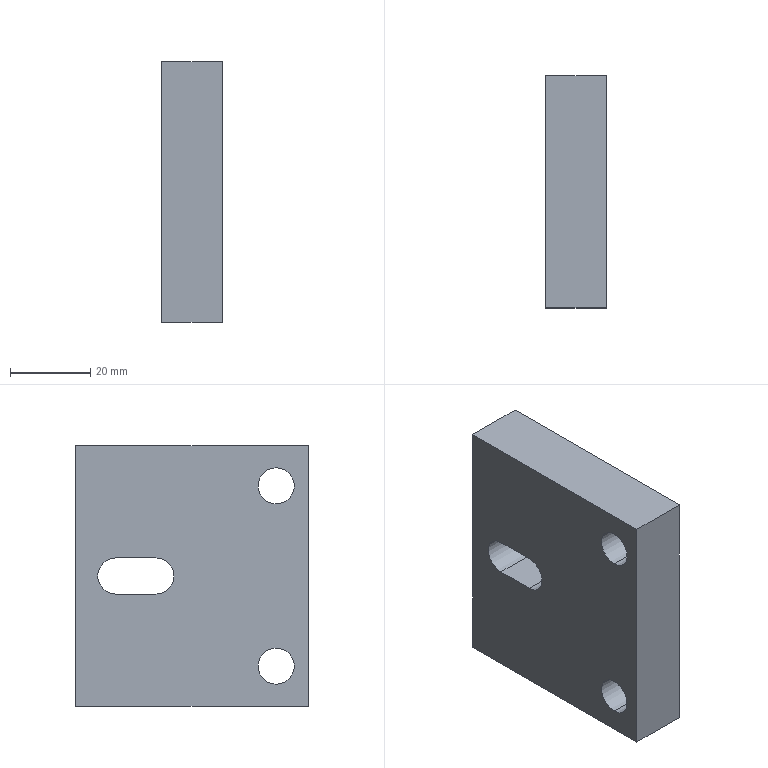Component | SolidWorks | TractionTensionPlate-2 | 1 solid | 14 faces | box 15 x 58 x 65 mm | volume 52337 mm3 | plane 8 | cylinder 6 | commonest cylinder face diameters 9 x6
build123d program:
from build123d import *

# Parameters (mm, degrees)
SKETCH1_W      = 65
SKETCH1_H      = 58
SKETCH1_R      = 4.5
EXTRUDE1_DEPTH = 15


with BuildPart() as part:
    # Sketch1 → Extrude1 (new body)
    with BuildSketch(Plane.XY):
        Rectangle(SKETCH1_W, SKETCH1_H)
        with Locations((-22.5, -21)):
            Circle(SKETCH1_R, mode=Mode.SUBTRACT)
        with Locations((22.5, -21)):
            Circle(SKETCH1_R, mode=Mode.SUBTRACT)
        with BuildLine():
            Line((-4.5, 19), (-4.5, 9))
            ThreePointArc((-4.5, 9), (0, 4.5), (4.5, 9))
            Line((4.5, 9), (4.5, 19))
            ThreePointArc((4.5, 19), (0, 23.5), (-4.5, 19))
        make_face(mode=Mode.SUBTRACT)
    extrude(amount=EXTRUDE1_DEPTH)


solid = part.part

# Placed as in the assembly
solid = solid.moved(Location((50.216, 516.983, 59.606), (0, 90, 0)))
STEP:
#1=CARTESIAN_POINT('',(2.568,19.527,1.638));
#2=VERTEX_POINT('',#1);
#3=CARTESIAN_POINT('',(2.568,19.527,1.284));
#4=VERTEX_POINT('',#3);
#5=CARTESIAN_POINT('',(2.568,19.527,1.461));
#6=DIRECTION('',(1.,0.,0.));
#7=DIRECTION('',(0.,0.,-1.));
#8=AXIS2_PLACEMENT_3D('',#5,#6,#7);
#9=CIRCLE('',#8,0.1772);
#10=EDGE_CURVE('',#2,#4,#9,.T.);
#11=ORIENTED_EDGE('',*,*,#10,.T.);
#12=CARTESIAN_POINT('',(1.977,19.527,1.284));
#13=VERTEX_POINT('',#12);
#14=CARTESIAN_POINT('',(2.568,19.527,1.284));
#15=DIRECTION('',(-1.,0.,0.));
#16=VECTOR('',#15,39.37);
#17=LINE('',#14,#16);
#18=EDGE_CURVE('',#4,#13,#17,.T.);
#19=ORIENTED_EDGE('',*,*,#18,.T.);
#20=CARTESIAN_POINT('',(1.977,19.527,1.638));
#21=VERTEX_POINT('',#20);
#22=CARTESIAN_POINT('',(1.977,19.527,1.461));
#23=DIRECTION('',(1.,0.,0.));
#24=DIRECTION('',(0.,0.,-1.));
#25=AXIS2_PLACEMENT_3D('',#22,#23,#24);
#26=CIRCLE('',#25,0.1772);
#27=EDGE_CURVE('',#21,#13,#26,.T.);
#28=ORIENTED_EDGE('',*,*,#27,.F.);
#29=CARTESIAN_POINT('',(2.568,19.527,1.638));
#30=DIRECTION('',(-1.,0.,0.));
#31=VECTOR('',#30,39.37);
#32=LINE('',#29,#31);
#33=EDGE_CURVE('',#2,#21,#32,.T.);
#34=ORIENTED_EDGE('',*,*,#33,.F.);
#35=EDGE_LOOP('',(#11,#19,#28,#34));
#36=FACE_OUTER_BOUND('',#35,.T.);
#37=CARTESIAN_POINT('',(2.568,19.527,1.461));
#38=DIRECTION('',(-1.,0.,0.));
#39=DIRECTION('',(0.,0.,1.));
#40=AXIS2_PLACEMENT_3D('',#37,#38,#39);
#41=CYLINDRICAL_SURFACE('',#40,0.1772);
#42=ADVANCED_FACE('',(#36),#41,.F.);
#43=CARTESIAN_POINT('',(2.568,19.527,3.41));
#44=VERTEX_POINT('',#43);
#45=CARTESIAN_POINT('',(2.568,19.527,3.055));
#46=VERTEX_POINT('',#45);
#47=CARTESIAN_POINT('',(2.568,19.527,3.233));
#48=DIRECTION('',(1.,0.,0.));
#49=DIRECTION('',(0.,0.,-1.));
#50=AXIS2_PLACEMENT_3D('',#47,#48,#49);
#51=CIRCLE('',#50,0.1772);
#52=EDGE_CURVE('',#44,#46,#51,.T.);
#53=ORIENTED_EDGE('',*,*,#52,.T.);
#54=CARTESIAN_POINT('',(1.977,19.527,3.055));
#55=VERTEX_POINT('',#54);
#56=CARTESIAN_POINT('',(2.568,19.527,3.055));
#57=DIRECTION('',(-1.,0.,0.));
#58=VECTOR('',#57,39.37);
#59=LINE('',#56,#58);
#60=EDGE_CURVE('',#46,#55,#59,.T.);
#61=ORIENTED_EDGE('',*,*,#60,.T.);
#62=CARTESIAN_POINT('',(1.977,19.527,3.41));
#63=VERTEX_POINT('',#62);
#64=CARTESIAN_POINT('',(1.977,19.527,3.233));
#65=DIRECTION('',(1.,0.,0.));
#66=DIRECTION('',(0.,0.,-1.));
#67=AXIS2_PLACEMENT_3D('',#64,#65,#66);
#68=CIRCLE('',#67,0.1772);
#69=EDGE_CURVE('',#63,#55,#68,.T.);
#70=ORIENTED_EDGE('',*,*,#69,.F.);
#71=CARTESIAN_POINT('',(2.568,19.527,3.41));
#72=DIRECTION('',(-1.,0.,0.));
#73=VECTOR('',#72,39.37);
#74=LINE('',#71,#73);
#75=EDGE_CURVE('',#44,#63,#74,.T.);
#76=ORIENTED_EDGE('',*,*,#75,.F.);
#77=EDGE_LOOP('',(#53,#61,#70,#76));
#78=FACE_OUTER_BOUND('',#77,.T.);
#79=CARTESIAN_POINT('',(2.568,19.527,3.233));
#80=DIRECTION('',(-1.,0.,0.));
#81=DIRECTION('',(0.,0.,1.));
#82=AXIS2_PLACEMENT_3D('',#79,#80,#81);
#83=CYLINDRICAL_SURFACE('',#82,0.1772);
#84=ADVANCED_FACE('',(#78),#83,.F.);
#85=ORIENTED_EDGE('',*,*,#52,.F.);
#86=CARTESIAN_POINT('',(2.568,19.527,3.233));
#87=DIRECTION('',(1.,0.,0.));
#88=DIRECTION('',(0.,0.,-1.));
#89=AXIS2_PLACEMENT_3D('',#86,#87,#88);
#90=CIRCLE('',#89,0.1772);
#91=EDGE_CURVE('',#46,#44,#90,.T.);
#92=ORIENTED_EDGE('',*,*,#91,.F.);
#93=EDGE_LOOP('',(#85,#92));
#94=FACE_BOUND('',#93,.T.);
#95=CARTESIAN_POINT('',(2.568,21.495,3.626));
#96=VERTEX_POINT('',#95);
#97=CARTESIAN_POINT('',(2.568,19.212,3.626));
#98=VERTEX_POINT('',#97);
#99=CARTESIAN_POINT('',(2.568,21.495,3.626));
#100=DIRECTION('',(0.,-1.,0.));
#101=VECTOR('',#100,39.37);
#102=LINE('',#99,#101);
#103=EDGE_CURVE('',#96,#98,#102,.T.);
#104=ORIENTED_EDGE('',*,*,#103,.T.);
#105=CARTESIAN_POINT('',(2.568,19.212,1.067));
#106=VERTEX_POINT('',#105);
#107=CARTESIAN_POINT('',(2.568,19.212,3.626));
#108=DIRECTION('',(0.,0.,-1.));
#109=VECTOR('',#108,39.37);
#110=LINE('',#107,#109);
#111=EDGE_CURVE('',#98,#106,#110,.T.);
#112=ORIENTED_EDGE('',*,*,#111,.T.);
#113=CARTESIAN_POINT('',(2.568,21.495,1.067));
#114=VERTEX_POINT('',#113);
#115=CARTESIAN_POINT('',(2.568,21.495,1.067));
#116=DIRECTION('',(0.,1.,0.));
#117=VECTOR('',#116,39.37);
#118=LINE('',#115,#117);
#119=EDGE_CURVE('',#106,#114,#118,.T.);
#120=ORIENTED_EDGE('',*,*,#119,.T.);
#121=CARTESIAN_POINT('',(2.568,21.495,3.626));
#122=DIRECTION('',(0.,0.,1.));
#123=VECTOR('',#122,39.37);
#124=LINE('',#121,#123);
#125=EDGE_CURVE('',#114,#96,#124,.T.);
#126=ORIENTED_EDGE('',*,*,#125,.T.);
#127=EDGE_LOOP('',(#104,#112,#120,#126));
#128=FACE_OUTER_BOUND('',#127,.T.);
#129=ORIENTED_EDGE('',*,*,#10,.F.);
#130=CARTESIAN_POINT('',(2.568,19.527,1.461));
#131=DIRECTION('',(1.,0.,0.));
#132=DIRECTION('',(0.,0.,-1.));
#133=AXIS2_PLACEMENT_3D('',#130,#131,#132);
#134=CIRCLE('',#133,0.1772);
#135=EDGE_CURVE('',#4,#2,#134,.T.);
#136=ORIENTED_EDGE('',*,*,#135,.F.);
#137=EDGE_LOOP('',(#129,#136));
#138=FACE_BOUND('',#137,.T.);
#139=CARTESIAN_POINT('',(2.568,21.102,2.524));
#140=VERTEX_POINT('',#139);
#141=CARTESIAN_POINT('',(2.568,20.708,2.524));
#142=VERTEX_POINT('',#141);
#143=CARTESIAN_POINT('',(2.568,21.102,2.524));
#144=DIRECTION('',(0.,-1.,0.));
#145=VECTOR('',#144,39.37);
#146=LINE('',#143,#145);
#147=EDGE_CURVE('',#140,#142,#146,.T.);
#148=ORIENTED_EDGE('',*,*,#147,.F.);
#149=CARTESIAN_POINT('',(2.568,21.102,2.17));
#150=VERTEX_POINT('',#149);
#151=CARTESIAN_POINT('',(2.568,21.102,2.347));
#152=DIRECTION('',(1.,0.,0.));
#153=DIRECTION('',(0.,0.,-1.));
#154=AXIS2_PLACEMENT_3D('',#151,#152,#153);
#155=CIRCLE('',#154,0.1772);
#156=EDGE_CURVE('',#150,#140,#155,.T.);
#157=ORIENTED_EDGE('',*,*,#156,.F.);
#158=CARTESIAN_POINT('',(2.568,20.708,2.17));
#159=VERTEX_POINT('',#158);
#160=CARTESIAN_POINT('',(2.568,21.102,2.17));
#161=DIRECTION('',(0.,1.,0.));
#162=VECTOR('',#161,39.37);
#163=LINE('',#160,#162);
#164=EDGE_CURVE('',#159,#150,#163,.T.);
#165=ORIENTED_EDGE('',*,*,#164,.F.);
#166=CARTESIAN_POINT('',(2.568,20.708,2.347));
#167=DIRECTION('',(1.,0.,0.));
#168=DIRECTION('',(0.,0.,-1.));
#169=AXIS2_PLACEMENT_3D('',#166,#167,#168);
#170=CIRCLE('',#169,0.1772);
#171=EDGE_CURVE('',#142,#159,#170,.T.);
#172=ORIENTED_EDGE('',*,*,#171,.F.);
#173=EDGE_LOOP('',(#148,#157,#165,#172));
#174=FACE_BOUND('',#173,.T.);
#175=CARTESIAN_POINT('',(2.568,19.212,3.626));
#176=DIRECTION('',(1.,0.,0.));
#177=DIRECTION('',(0.,0.,-1.));
#178=AXIS2_PLACEMENT_3D('',#175,#176,#177);
#179=PLANE('',#178);
#180=ADVANCED_FACE('',(#94,#128,#138,#174),#179,.T.);
#181=ORIENTED_EDGE('',*,*,#27,.T.);
#182=CARTESIAN_POINT('',(1.977,19.527,1.461));
#183=DIRECTION('',(1.,0.,0.));
#184=DIRECTION('',(0.,0.,-1.));
#185=AXIS2_PLACEMENT_3D('',#182,#183,#184);
#186=CIRCLE('',#185,0.1772);
#187=EDGE_CURVE('',#13,#21,#186,.T.);
#188=ORIENTED_EDGE('',*,*,#187,.T.);
#189=EDGE_LOOP('',(#181,#188));
#190=FACE_BOUND('',#189,.T.);
#191=ORIENTED_EDGE('',*,*,#69,.T.);
#192=CARTESIAN_POINT('',(1.977,19.527,3.233));
#193=DIRECTION('',(1.,0.,0.));
#194=DIRECTION('',(0.,0.,-1.));
#195=AXIS2_PLACEMENT_3D('',#192,#193,#194);
#196=CIRCLE('',#195,0.1772);
#197=EDGE_CURVE('',#55,#63,#196,.T.);
#198=ORIENTED_EDGE('',*,*,#197,.T.);
#199=EDGE_LOOP('',(#191,#198));
#200=FACE_BOUND('',#199,.T.);
#201=CARTESIAN_POINT('',(1.977,21.495,3.626));
#202=VERTEX_POINT('',#201);
#203=CARTESIAN_POINT('',(1.977,19.212,3.626));
#204=VERTEX_POINT('',#203);
#205=CARTESIAN_POINT('',(1.977,21.495,3.626));
#206=DIRECTION('',(0.,-1.,0.));
#207=VECTOR('',#206,39.37);
#208=LINE('',#205,#207);
#209=EDGE_CURVE('',#202,#204,#208,.T.);
#210=ORIENTED_EDGE('',*,*,#209,.F.);
#211=CARTESIAN_POINT('',(1.977,21.495,1.067));
#212=VERTEX_POINT('',#211);
#213=CARTESIAN_POINT('',(1.977,21.495,3.626));
#214=DIRECTION('',(0.,0.,1.));
#215=VECTOR('',#214,39.37);
#216=LINE('',#213,#215);
#217=EDGE_CURVE('',#212,#202,#216,.T.);
#218=ORIENTED_EDGE('',*,*,#217,.F.);
#219=CARTESIAN_POINT('',(1.977,19.212,1.067));
#220=VERTEX_POINT('',#219);
#221=CARTESIAN_POINT('',(1.977,21.495,1.067));
#222=DIRECTION('',(0.,1.,0.));
#223=VECTOR('',#222,39.37);
#224=LINE('',#221,#223);
#225=EDGE_CURVE('',#220,#212,#224,.T.);
#226=ORIENTED_EDGE('',*,*,#225,.F.);
#227=CARTESIAN_POINT('',(1.977,19.212,3.626));
#228=DIRECTION('',(0.,0.,-1.));
#229=VECTOR('',#228,39.37);
#230=LINE('',#227,#229);
#231=EDGE_CURVE('',#204,#220,#230,.T.);
#232=ORIENTED_EDGE('',*,*,#231,.F.);
#233=EDGE_LOOP('',(#210,#218,#226,#232));
#234=FACE_OUTER_BOUND('',#233,.T.);
#235=CARTESIAN_POINT('',(1.977,21.102,2.17));
#236=VERTEX_POINT('',#235);
#237=CARTESIAN_POINT('',(1.977,21.102,2.524));
#238=VERTEX_POINT('',#237);
#239=CARTESIAN_POINT('',(1.977,21.102,2.347));
#240=DIRECTION('',(1.,0.,0.));
#241=DIRECTION('',(0.,0.,-1.));
#242=AXIS2_PLACEMENT_3D('',#239,#240,#241);
#243=CIRCLE('',#242,0.1772);
#244=EDGE_CURVE('',#236,#238,#243,.T.);
#245=ORIENTED_EDGE('',*,*,#244,.T.);
#246=CARTESIAN_POINT('',(1.977,20.708,2.524));
#247=VERTEX_POINT('',#246);
#248=CARTESIAN_POINT('',(1.977,21.102,2.524));
#249=DIRECTION('',(0.,-1.,0.));
#250=VECTOR('',#249,39.37);
#251=LINE('',#248,#250);
#252=EDGE_CURVE('',#238,#247,#251,.T.);
#253=ORIENTED_EDGE('',*,*,#252,.T.);
#254=CARTESIAN_POINT('',(1.977,20.708,2.17));
#255=VERTEX_POINT('',#254);
#256=CARTESIAN_POINT('',(1.977,20.708,2.347));
#257=DIRECTION('',(1.,0.,0.));
#258=DIRECTION('',(0.,0.,-1.));
#259=AXIS2_PLACEMENT_3D('',#256,#257,#258);
#260=CIRCLE('',#259,0.1772);
#261=EDGE_CURVE('',#247,#255,#260,.T.);
#262=ORIENTED_EDGE('',*,*,#261,.T.);
#263=CARTESIAN_POINT('',(1.977,21.102,2.17));
#264=DIRECTION('',(0.,1.,0.));
#265=VECTOR('',#264,39.37);
#266=LINE('',#263,#265);
#267=EDGE_CURVE('',#255,#236,#266,.T.);
#268=ORIENTED_EDGE('',*,*,#267,.T.);
#269=EDGE_LOOP('',(#245,#253,#262,#268));
#270=FACE_BOUND('',#269,.T.);
#271=CARTESIAN_POINT('',(1.977,19.212,3.626));
#272=DIRECTION('',(1.,0.,0.));
#273=DIRECTION('',(0.,0.,-1.));
#274=AXIS2_PLACEMENT_3D('',#271,#272,#273);
#275=PLANE('',#274);
#276=ADVANCED_FACE('',(#190,#200,#234,#270),#275,.F.);
#277=ORIENTED_EDGE('',*,*,#209,.T.);
#278=CARTESIAN_POINT('',(2.568,19.212,3.626));
#279=DIRECTION('',(-1.,0.,0.));
#280=VECTOR('',#279,39.37);
#281=LINE('',#278,#280);
#282=EDGE_CURVE('',#98,#204,#281,.T.);
#283=ORIENTED_EDGE('',*,*,#282,.F.);
#284=ORIENTED_EDGE('',*,*,#103,.F.);
#285=CARTESIAN_POINT('',(2.568,21.495,3.626));
#286=DIRECTION('',(-1.,0.,0.));
#287=VECTOR('',#286,39.37);
#288=LINE('',#285,#287);
#289=EDGE_CURVE('',#96,#202,#288,.T.);
#290=ORIENTED_EDGE('',*,*,#289,.T.);
#291=EDGE_LOOP('',(#277,#283,#284,#290));
#292=FACE_OUTER_BOUND('',#291,.T.);
#293=CARTESIAN_POINT('',(2.568,21.495,3.626));
#294=DIRECTION('',(0.,0.,-1.));
#295=DIRECTION('',(-1.,0.,0.));
#296=AXIS2_PLACEMENT_3D('',#293,#294,#295);
#297=PLANE('',#296);
#298=ADVANCED_FACE('',(#292),#297,.F.);
#299=ORIENTED_EDGE('',*,*,#231,.T.);
#300=CARTESIAN_POINT('',(2.568,19.212,1.067));
#301=DIRECTION('',(-1.,0.,0.));
#302=VECTOR('',#301,39.37);
#303=LINE('',#300,#302);
#304=EDGE_CURVE('',#106,#220,#303,.T.);
#305=ORIENTED_EDGE('',*,*,#304,.F.);
#306=ORIENTED_EDGE('',*,*,#111,.F.);
#307=ORIENTED_EDGE('',*,*,#282,.T.);
#308=EDGE_LOOP('',(#299,#305,#306,#307));
#309=FACE_OUTER_BOUND('',#308,.T.);
#310=CARTESIAN_POINT('',(2.568,19.212,3.626));
#311=DIRECTION('',(0.,1.,0.));
#312=DIRECTION('',(1.,0.,0.));
#313=AXIS2_PLACEMENT_3D('',#310,#311,#312);
#314=PLANE('',#313);
#315=ADVANCED_FACE('',(#309),#314,.F.);
#316=ORIENTED_EDGE('',*,*,#225,.T.);
#317=CARTESIAN_POINT('',(2.568,21.495,1.067));
#318=DIRECTION('',(-1.,0.,0.));
#319=VECTOR('',#318,39.37);
#320=LINE('',#317,#319);
#321=EDGE_CURVE('',#114,#212,#320,.T.);
#322=ORIENTED_EDGE('',*,*,#321,.F.);
#323=ORIENTED_EDGE('',*,*,#119,.F.);
#324=ORIENTED_EDGE('',*,*,#304,.T.);
#325=EDGE_LOOP('',(#316,#322,#323,#324));
#326=FACE_OUTER_BOUND('',#325,.T.);
#327=CARTESIAN_POINT('',(2.568,21.495,1.067));
#328=DIRECTION('',(0.,0.,1.));
#329=DIRECTION('',(1.,0.,0.));
#330=AXIS2_PLACEMENT_3D('',#327,#328,#329);
#331=PLANE('',#330);
#332=ADVANCED_FACE('',(#326),#331,.F.);
#333=ORIENTED_EDGE('',*,*,#217,.T.);
#334=ORIENTED_EDGE('',*,*,#289,.F.);
#335=ORIENTED_EDGE('',*,*,#125,.F.);
#336=ORIENTED_EDGE('',*,*,#321,.T.);
#337=EDGE_LOOP('',(#333,#334,#335,#336));
#338=FACE_OUTER_BOUND('',#337,.T.);
#339=CARTESIAN_POINT('',(2.568,21.495,3.626));
#340=DIRECTION('',(0.,-1.,0.));
#341=DIRECTION('',(-1.,0.,0.));
#342=AXIS2_PLACEMENT_3D('',#339,#340,#341);
#343=PLANE('',#342);
#344=ADVANCED_FACE('',(#338),#343,.F.);
#345=ORIENTED_EDGE('',*,*,#60,.F.);
#346=ORIENTED_EDGE('',*,*,#91,.T.);
#347=ORIENTED_EDGE('',*,*,#75,.T.);
#348=ORIENTED_EDGE('',*,*,#197,.F.);
#349=EDGE_LOOP('',(#345,#346,#347,#348));
#350=FACE_OUTER_BOUND('',#349,.T.);
#351=CARTESIAN_POINT('',(2.568,19.527,3.233));
#352=DIRECTION('',(-1.,0.,0.));
#353=DIRECTION('',(0.,0.,1.));
#354=AXIS2_PLACEMENT_3D('',#351,#352,#353);
#355=CYLINDRICAL_SURFACE('',#354,0.1772);
#356=ADVANCED_FACE('',(#350),#355,.F.);
#357=ORIENTED_EDGE('',*,*,#18,.F.);
#358=ORIENTED_EDGE('',*,*,#135,.T.);
#359=ORIENTED_EDGE('',*,*,#33,.T.);
#360=ORIENTED_EDGE('',*,*,#187,.F.);
#361=EDGE_LOOP('',(#357,#358,#359,#360));
#362=FACE_OUTER_BOUND('',#361,.T.);
#363=CARTESIAN_POINT('',(2.568,19.527,1.461));
#364=DIRECTION('',(-1.,0.,0.));
#365=DIRECTION('',(0.,0.,1.));
#366=AXIS2_PLACEMENT_3D('',#363,#364,#365);
#367=CYLINDRICAL_SURFACE('',#366,0.1772);
#368=ADVANCED_FACE('',(#362),#367,.F.);
#369=ORIENTED_EDGE('',*,*,#244,.F.);
#370=CARTESIAN_POINT('',(2.568,21.102,2.17));
#371=DIRECTION('',(-1.,0.,0.));
#372=VECTOR('',#371,39.37);
#373=LINE('',#370,#372);
#374=EDGE_CURVE('',#150,#236,#373,.T.);
#375=ORIENTED_EDGE('',*,*,#374,.F.);
#376=ORIENTED_EDGE('',*,*,#156,.T.);
#377=CARTESIAN_POINT('',(2.568,21.102,2.524));
#378=DIRECTION('',(-1.,0.,0.));
#379=VECTOR('',#378,39.37);
#380=LINE('',#377,#379);
#381=EDGE_CURVE('',#140,#238,#380,.T.);
#382=ORIENTED_EDGE('',*,*,#381,.T.);
#383=EDGE_LOOP('',(#369,#375,#376,#382));
#384=FACE_OUTER_BOUND('',#383,.T.);
#385=CARTESIAN_POINT('',(2.568,21.102,2.347));
#386=DIRECTION('',(-1.,0.,0.));
#387=DIRECTION('',(0.,0.,1.));
#388=AXIS2_PLACEMENT_3D('',#385,#386,#387);
#389=CYLINDRICAL_SURFACE('',#388,0.1772);
#390=ADVANCED_FACE('',(#384),#389,.F.);
#391=ORIENTED_EDGE('',*,*,#252,.F.);
#392=ORIENTED_EDGE('',*,*,#381,.F.);
#393=ORIENTED_EDGE('',*,*,#147,.T.);
#394=CARTESIAN_POINT('',(2.568,20.708,2.524));
#395=DIRECTION('',(-1.,0.,0.));
#396=VECTOR('',#395,39.37);
#397=LINE('',#394,#396);
#398=EDGE_CURVE('',#142,#247,#397,.T.);
#399=ORIENTED_EDGE('',*,*,#398,.T.);
#400=EDGE_LOOP('',(#391,#392,#393,#399));
#401=FACE_OUTER_BOUND('',#400,.T.);
#402=CARTESIAN_POINT('',(2.568,21.102,2.524));
#403=DIRECTION('',(0.,0.,-1.));
#404=DIRECTION('',(-1.,0.,0.));
#405=AXIS2_PLACEMENT_3D('',#402,#403,#404);
#406=PLANE('',#405);
#407=ADVANCED_FACE('',(#401),#406,.T.);
#408=ORIENTED_EDGE('',*,*,#261,.F.);
#409=ORIENTED_EDGE('',*,*,#398,.F.);
#410=ORIENTED_EDGE('',*,*,#171,.T.);
#411=CARTESIAN_POINT('',(2.568,20.708,2.17));
#412=DIRECTION('',(-1.,0.,0.));
#413=VECTOR('',#412,39.37);
#414=LINE('',#411,#413);
#415=EDGE_CURVE('',#159,#255,#414,.T.);
#416=ORIENTED_EDGE('',*,*,#415,.T.);
#417=EDGE_LOOP('',(#408,#409,#410,#416));
#418=FACE_OUTER_BOUND('',#417,.T.);
#419=CARTESIAN_POINT('',(2.568,20.708,2.347));
#420=DIRECTION('',(-1.,0.,0.));
#421=DIRECTION('',(0.,0.,1.));
#422=AXIS2_PLACEMENT_3D('',#419,#420,#421);
#423=CYLINDRICAL_SURFACE('',#422,0.1772);
#424=ADVANCED_FACE('',(#418),#423,.F.);
#425=ORIENTED_EDGE('',*,*,#267,.F.);
#426=ORIENTED_EDGE('',*,*,#415,.F.);
#427=ORIENTED_EDGE('',*,*,#164,.T.);
#428=ORIENTED_EDGE('',*,*,#374,.T.);
#429=EDGE_LOOP('',(#425,#426,#427,#428));
#430=FACE_OUTER_BOUND('',#429,.T.);
#431=CARTESIAN_POINT('',(2.568,21.102,2.17));
#432=DIRECTION('',(0.,-0.,1.));
#433=DIRECTION('',(0.,-1.,-0.));
#434=AXIS2_PLACEMENT_3D('',#431,#432,#433);
#435=PLANE('',#434);
#436=ADVANCED_FACE('',(#430),#435,.T.);
#437=CLOSED_SHELL('',(#42,#84,#180,#276,#298,#315,#332,#344,#356,#368,#390,#407,#424,#436));
#438=MANIFOLD_SOLID_BREP('',#437);
#439=CARTESIAN_POINT('',(0.,0.,0.));
#440=DIRECTION('',(0.,0.,1.));
#441=DIRECTION('',(1.,0.,0.));
#442=AXIS2_PLACEMENT_3D('',#439,#440,#441);
#443=(LENGTH_UNIT()NAMED_UNIT(*)SI_UNIT($,.METRE.));
#444=LENGTH_MEASURE_WITH_UNIT(LENGTH_MEASURE(0.0254),#443);
#445=DIMENSIONAL_EXPONENTS(1.,0.,0.,0.,0.,0.,0.);
#446=(CONVERSION_BASED_UNIT('',#444)LENGTH_UNIT()NAMED_UNIT(#445));
#447=UNCERTAINTY_MEASURE_WITH_UNIT(LENGTH_MEASURE(0.00001),#446,'','');
#448=(NAMED_UNIT(*)PLANE_ANGLE_UNIT()SI_UNIT($,.RADIAN.));
#449=(NAMED_UNIT(*)SI_UNIT($,.STERADIAN.)SOLID_ANGLE_UNIT());
#450=(GEOMETRIC_REPRESENTATION_CONTEXT(3)GLOBAL_UNCERTAINTY_ASSIGNED_CONTEXT((#447))GLOBAL_UNIT_ASSIGNED_CONTEXT((#446,#448,#449))REPRESENTATION_CONTEXT('',''));
#451=ADVANCED_BREP_SHAPE_REPRESENTATION('',(#438,#442),#450);
#452=COLOUR_RGB('',0.7922,0.8196,0.9333);
#453=FILL_AREA_STYLE_COLOUR('',#452);
#454=FILL_AREA_STYLE('',(#453));
#455=SURFACE_STYLE_FILL_AREA(#454);
#456=SURFACE_SIDE_STYLE('',(#455));
#457=SURFACE_STYLE_USAGE(.BOTH.,#456);
#458=PRESENTATION_STYLE_ASSIGNMENT((#457));
#459=STYLED_ITEM('',(#458),#438);
#460=(LENGTH_UNIT()NAMED_UNIT(*)SI_UNIT($,.METRE.));
#461=LENGTH_MEASURE_WITH_UNIT(LENGTH_MEASURE(0.0254),#460);
#462=DIMENSIONAL_EXPONENTS(1.,0.,0.,0.,0.,0.,0.);
#463=(CONVERSION_BASED_UNIT('',#461)LENGTH_UNIT()NAMED_UNIT(#462));
#464=UNCERTAINTY_MEASURE_WITH_UNIT(LENGTH_MEASURE(0.00001),#463,'','');
#465=(NAMED_UNIT(*)PLANE_ANGLE_UNIT()SI_UNIT($,.RADIAN.));
#466=(NAMED_UNIT(*)SI_UNIT($,.STERADIAN.)SOLID_ANGLE_UNIT());
#467=(GEOMETRIC_REPRESENTATION_CONTEXT(3)GLOBAL_UNCERTAINTY_ASSIGNED_CONTEXT((#464))GLOBAL_UNIT_ASSIGNED_CONTEXT((#463,#465,#466))REPRESENTATION_CONTEXT('',''));
#468=MECHANICAL_DESIGN_GEOMETRIC_PRESENTATION_REPRESENTATION('',(#459),#467);
#469=PRESENTATION_LAYER_ASSIGNMENT('','',(#459));